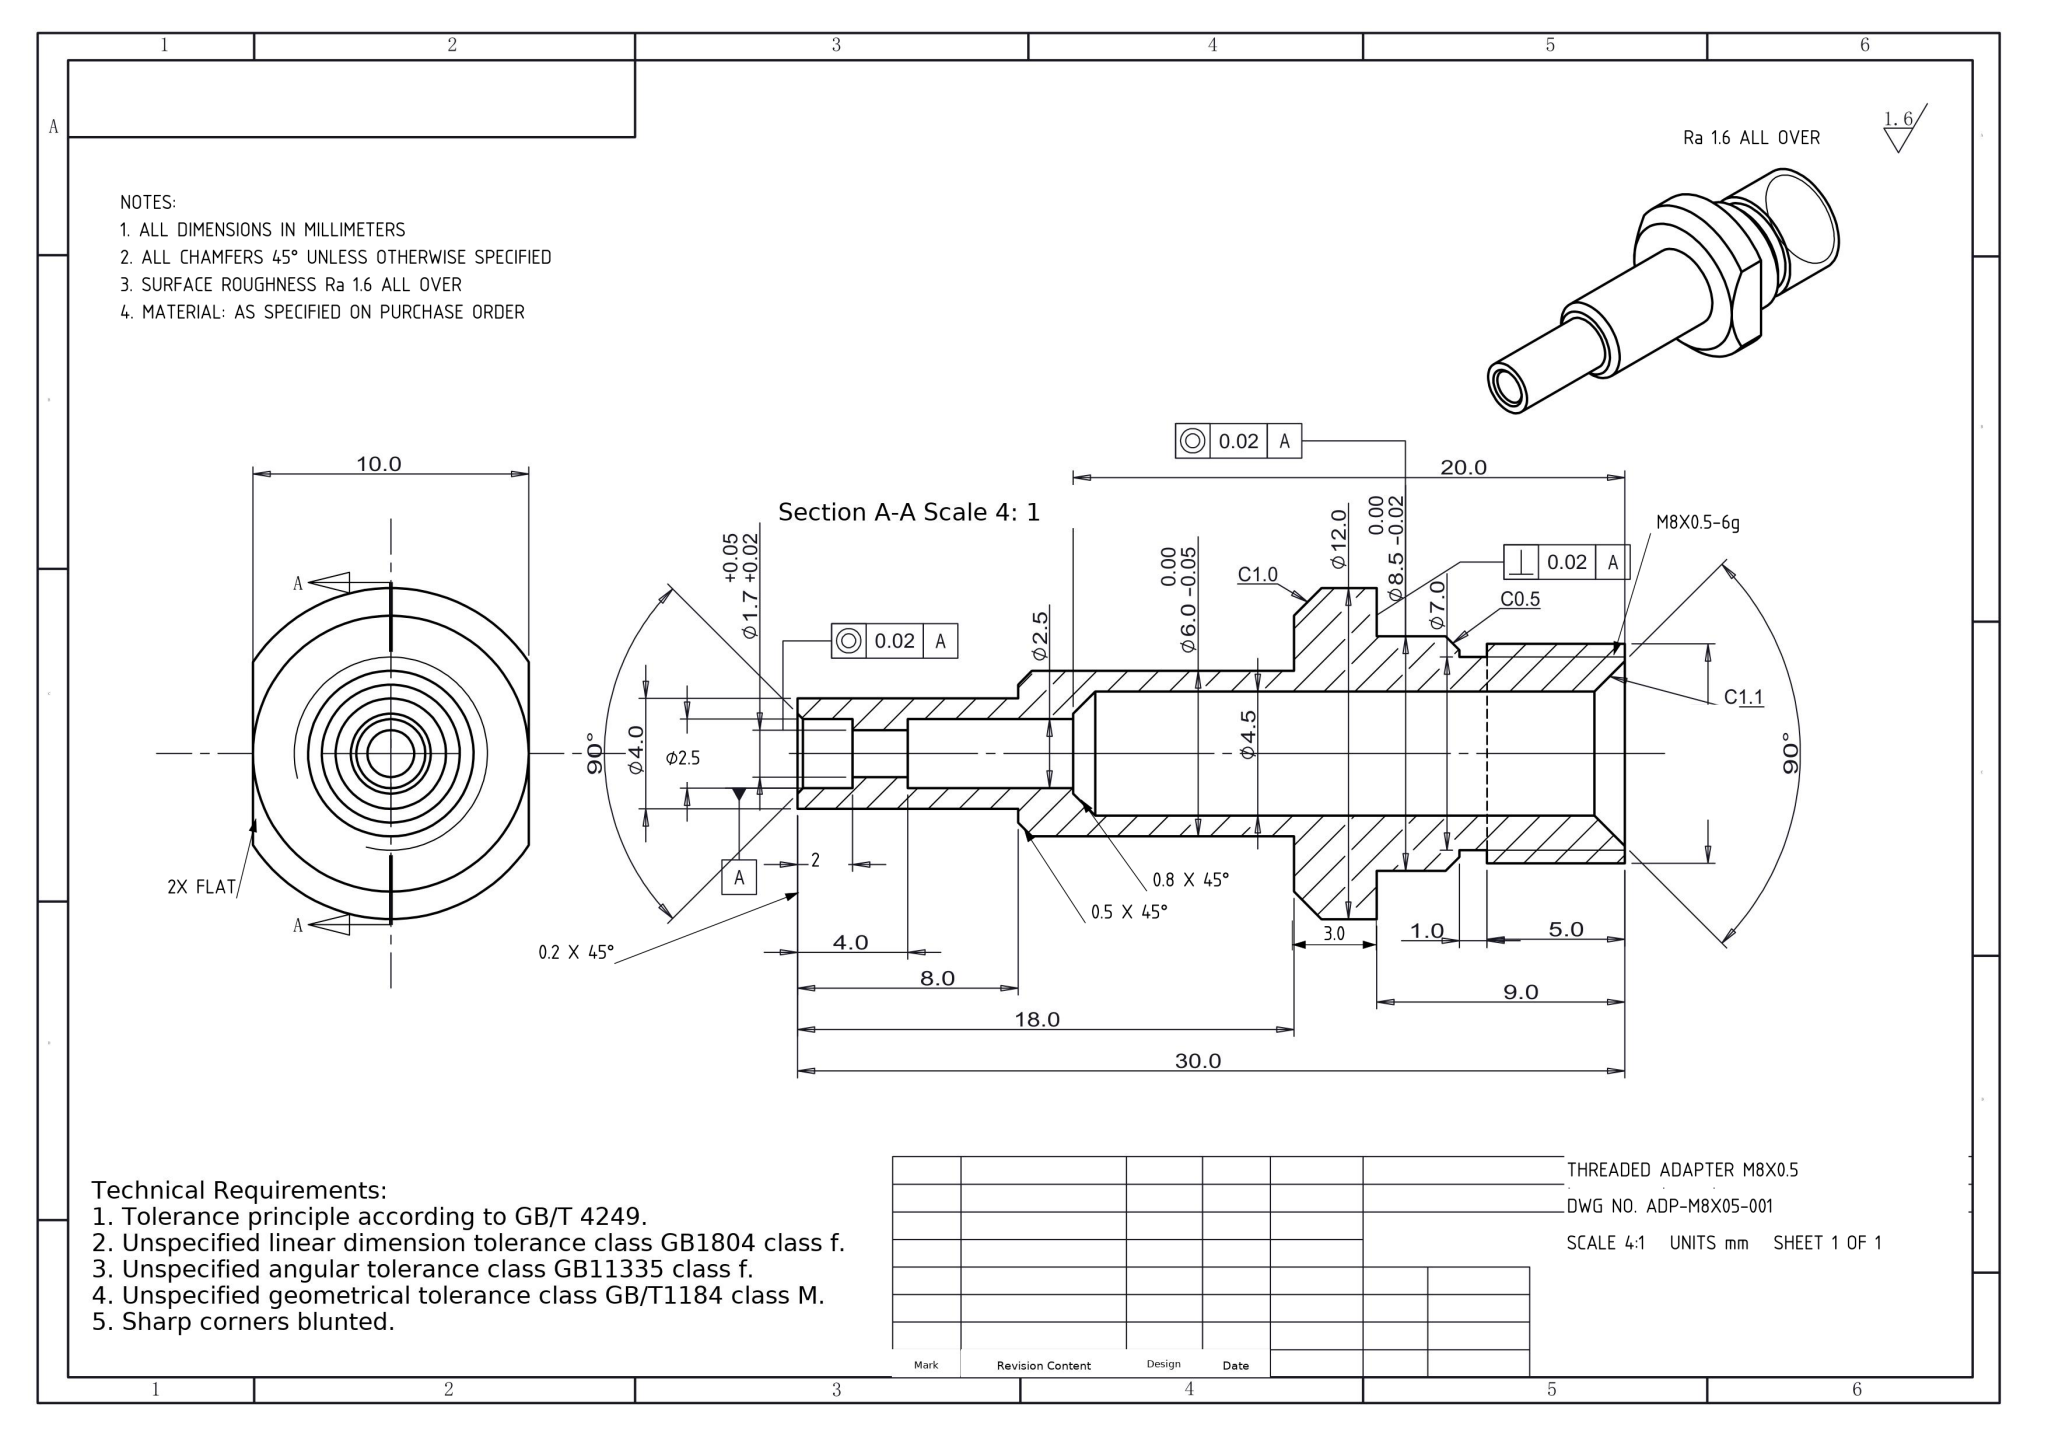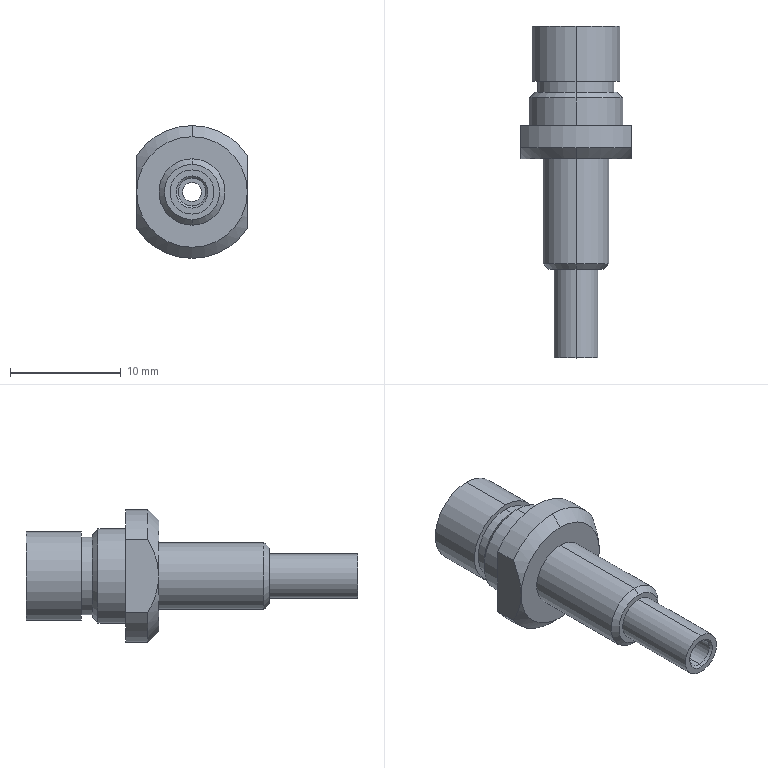Part | NX | mm | 1 solid | 46 faces | box 10 x 30 x 12 mm | volume 767 mm3 | cylinder 21 | cone 13 | plane 12 | commonest cylinder face diameters 2.5 x4 12 x3 4 x2 4.5 x2 1.7 x2 7 x2 7.96 x2 8.5 x2